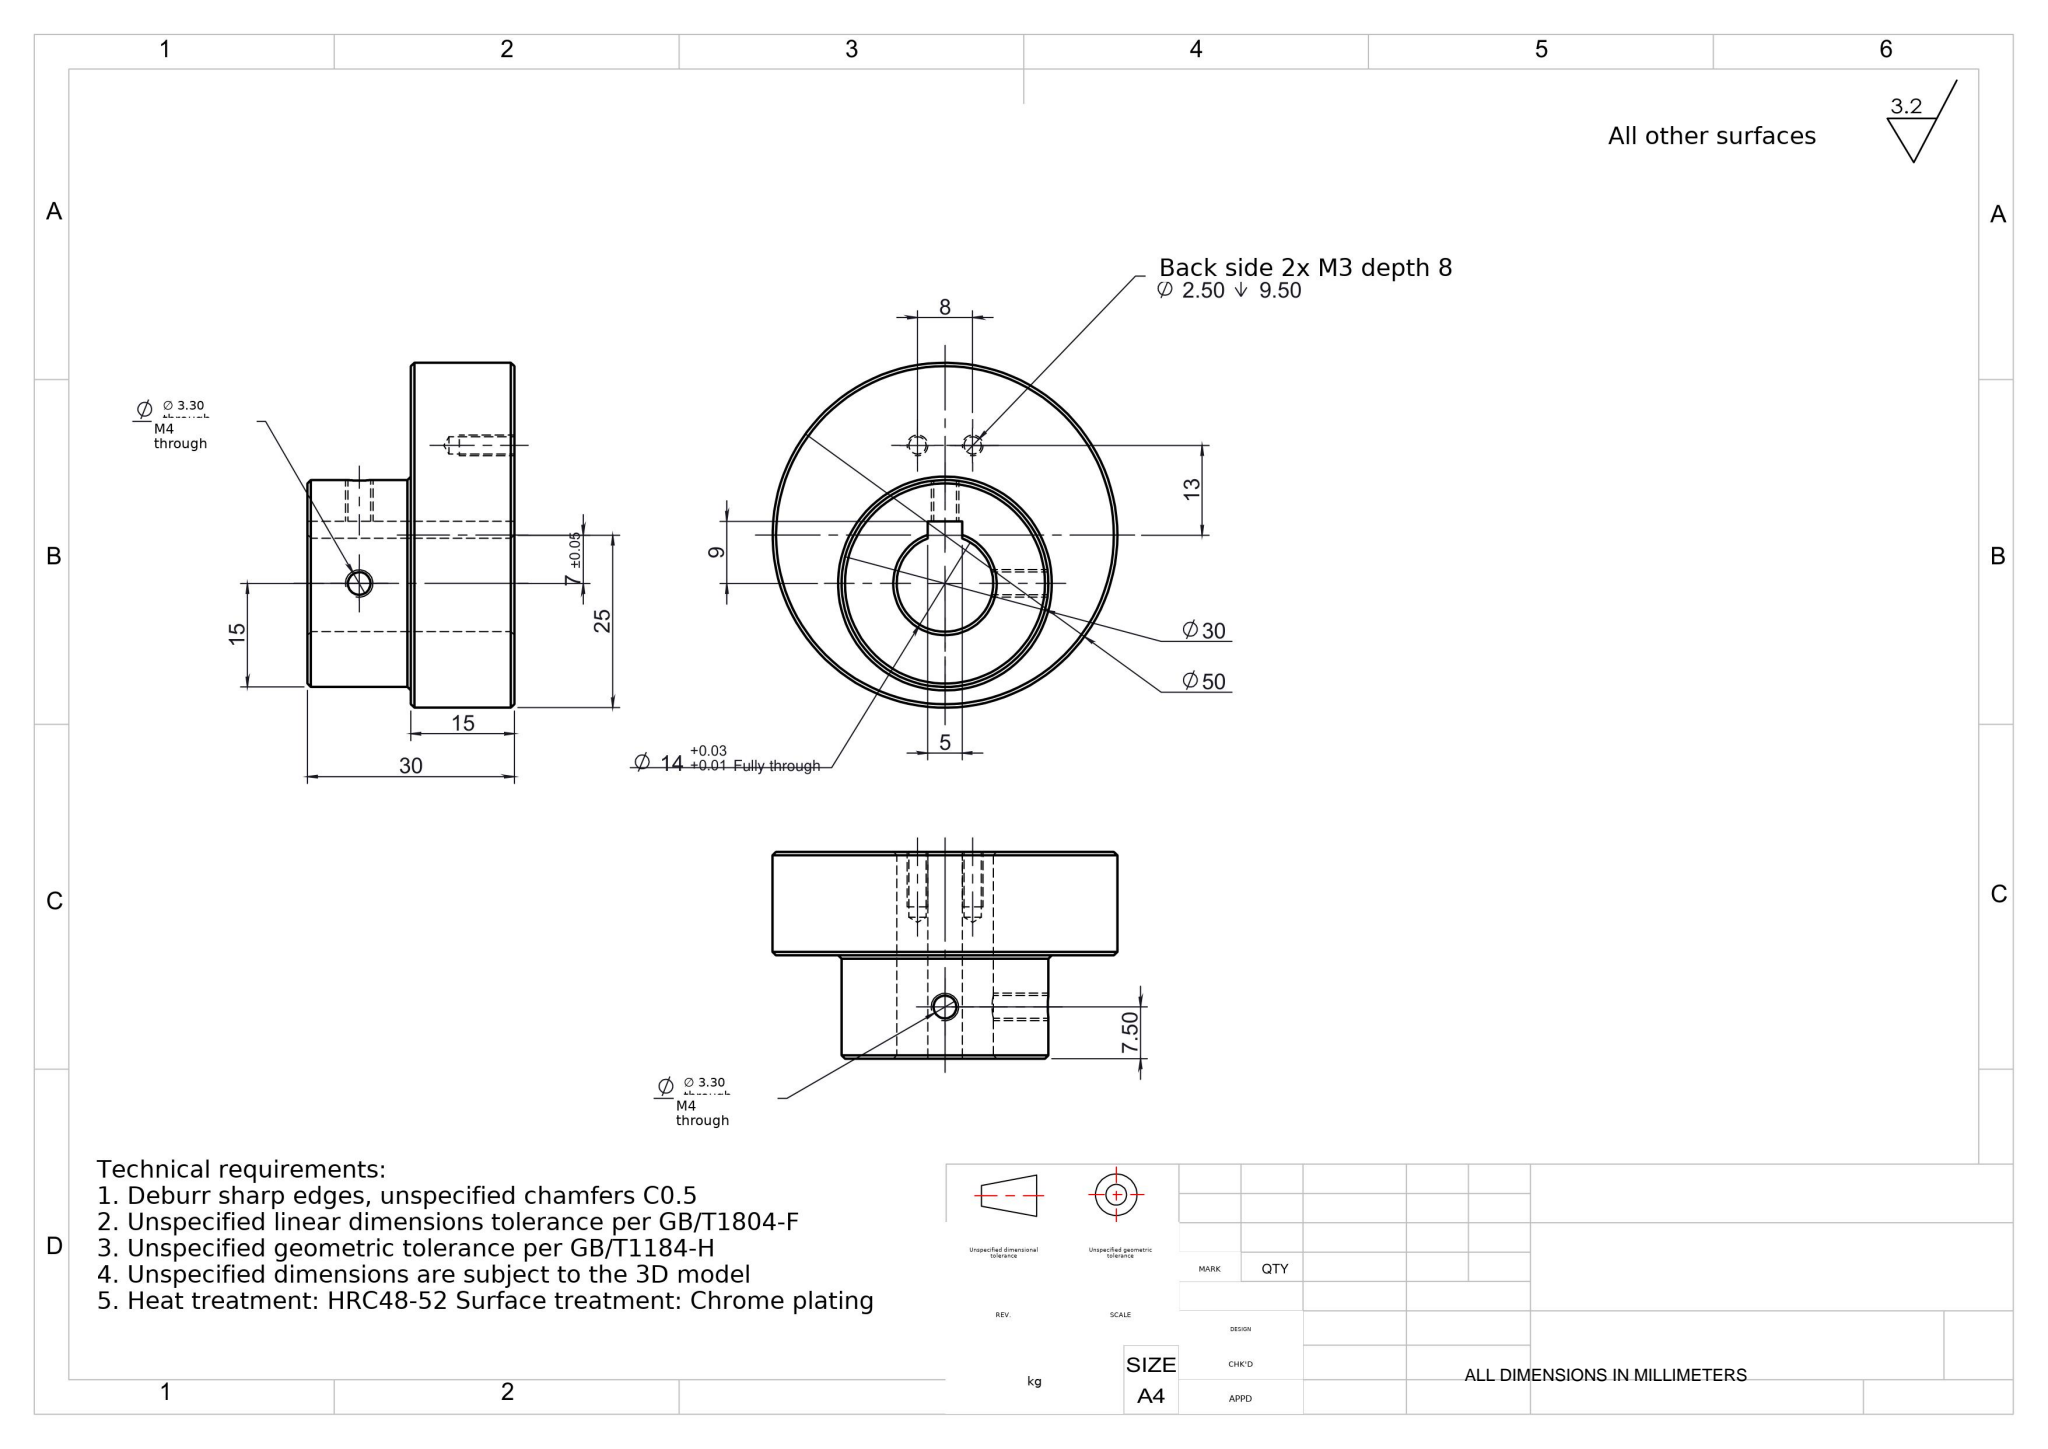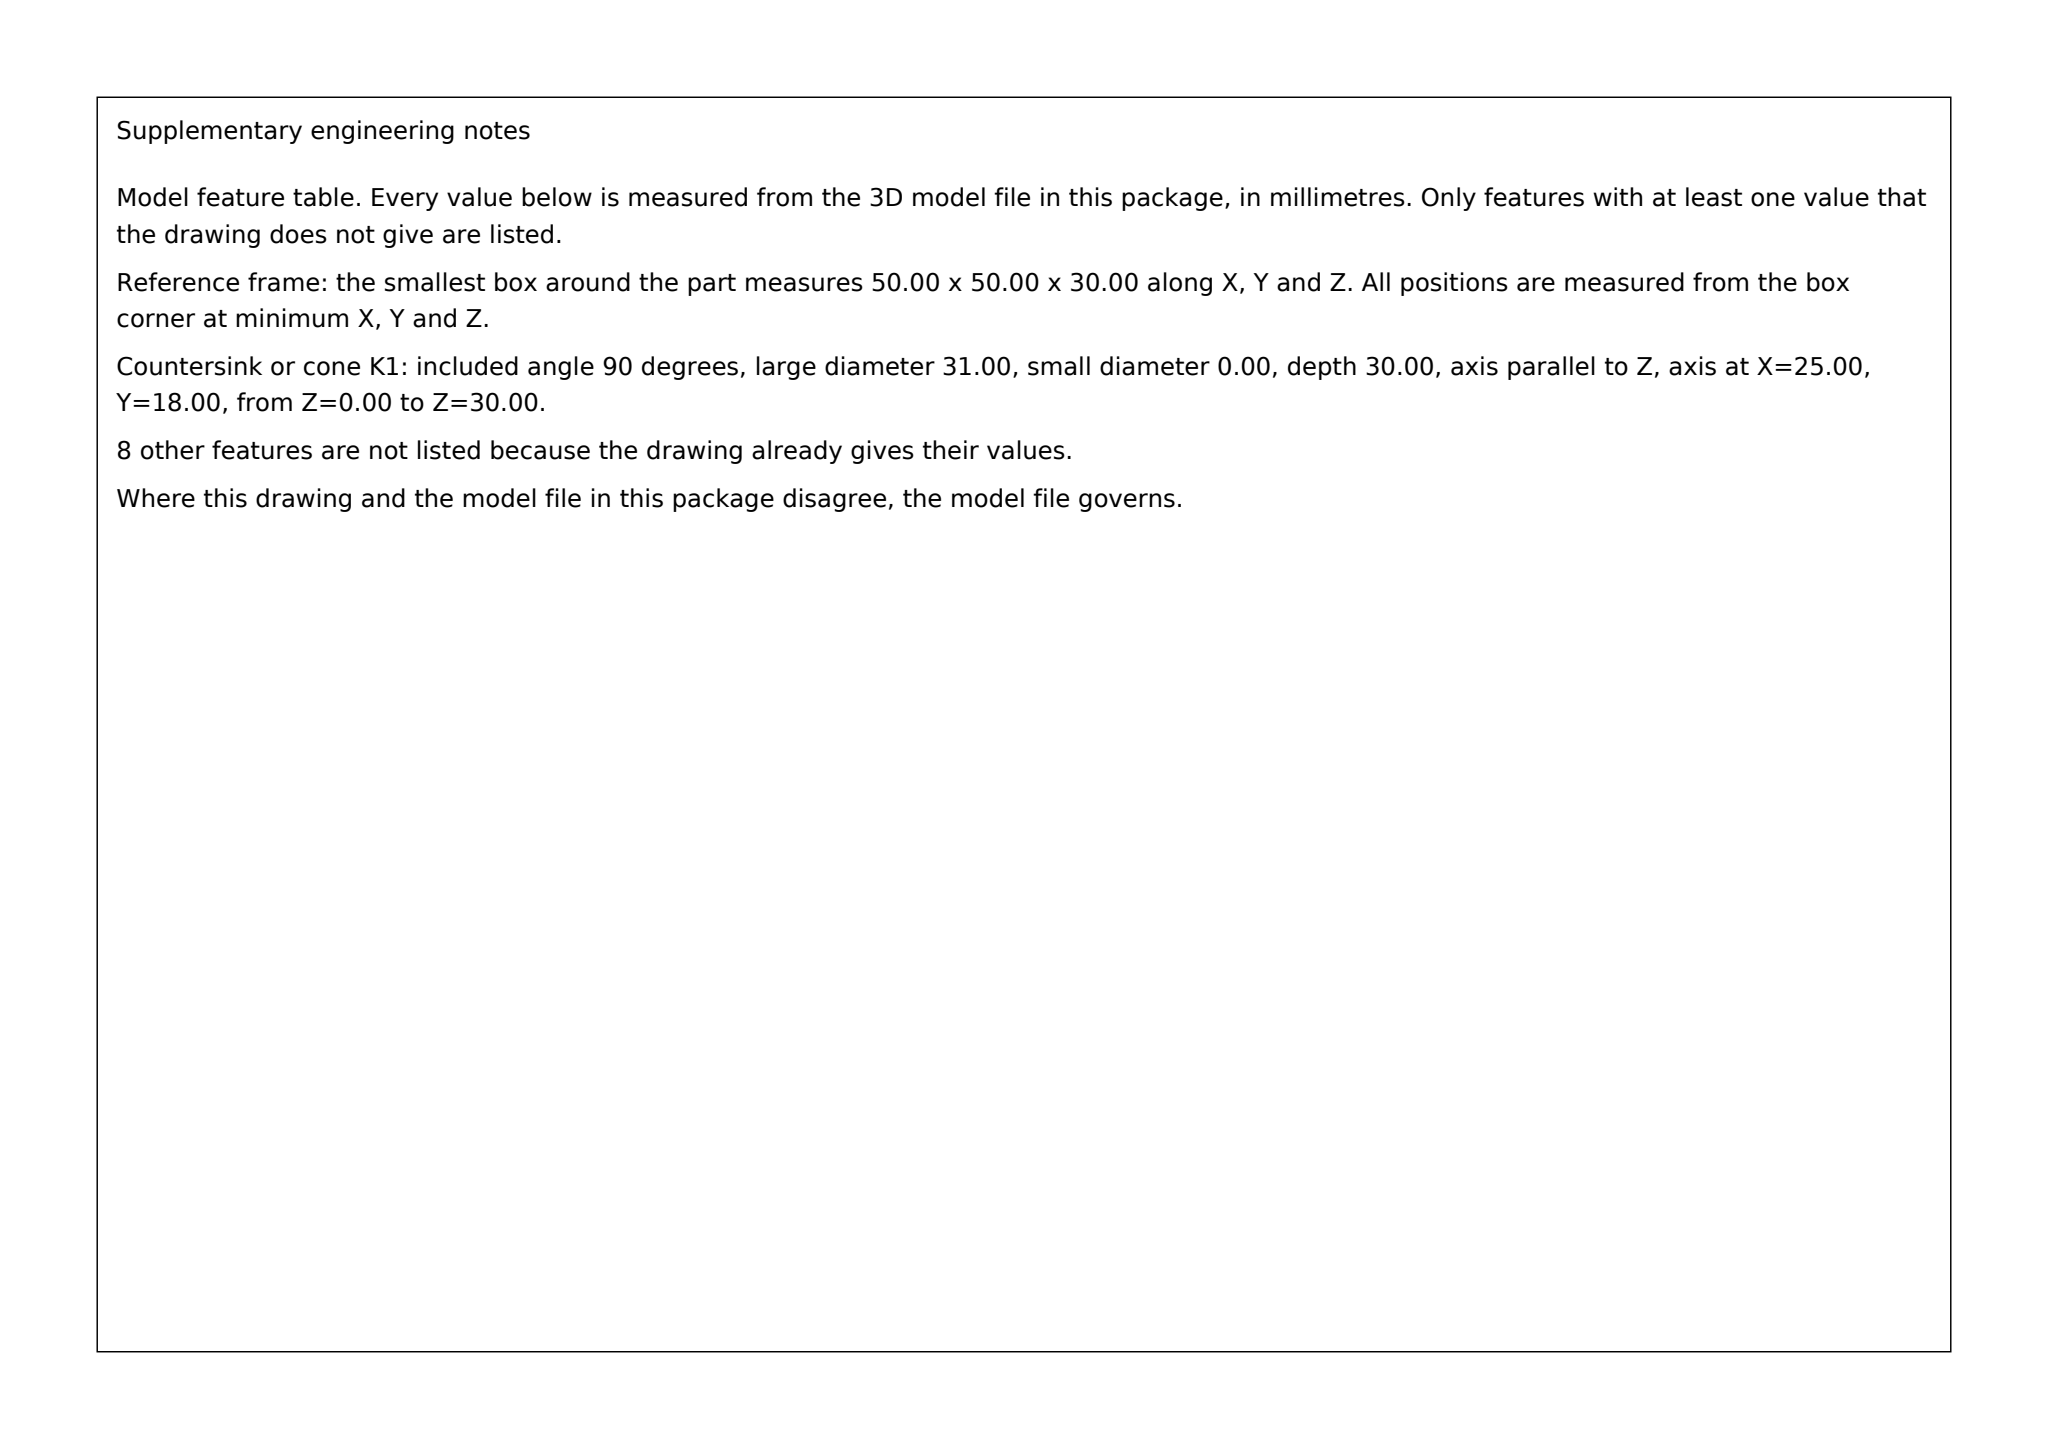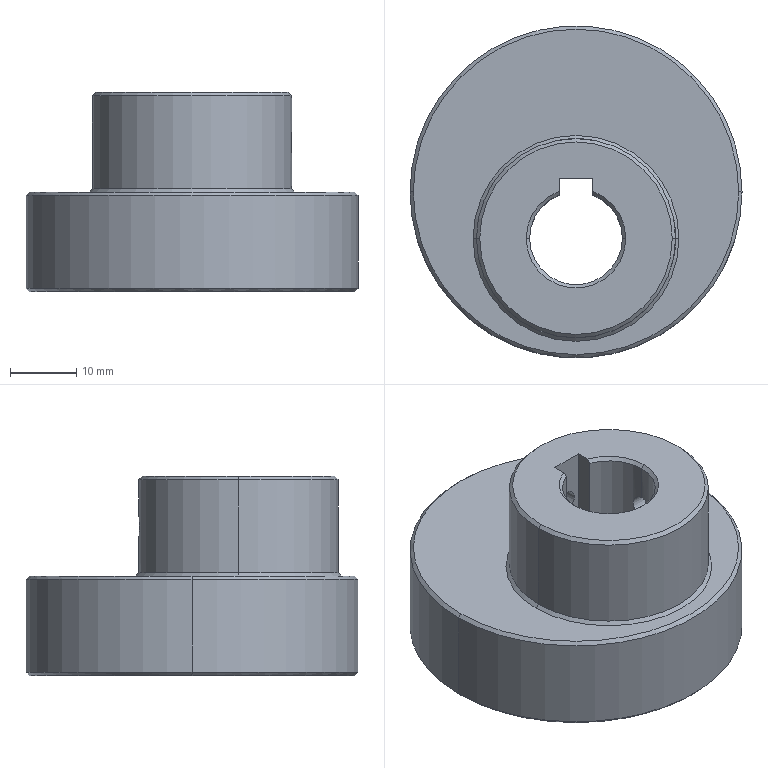Part | SolidWorks | mm | 1 solid | 39 faces | box 50 x 50 x 30 mm | volume 34850 mm3 | cone 18 | cylinder 15 | plane 6 | commonest cylinder face diameters 3.3 x4 2.5 x4 14 x3 30 x2 50 x2
build123d program:
from build123d import *

# Parameters (mm, degrees)
SKETCH1_R                  = 25
BOSS_EXTRUDE1_DEPTH        = 15
F_14_0_14_DIAMETER_HOLE1_D = 14
CHAMFER2_SIZE              = 0.5
M3_TAPPED_HOLE1_D          = 2.5
M3_TAPPED_HOLE1_DEPTH      = 9.5
M3_TAPPED_HOLE1_TIP        = 0.7511
SKETCH15_R                 = 47.133
SKETCH15_R_2               = 15
CUT_EXTRUDE3_DEPTH         = 15
CHAMFER1_SIZE              = 0.5
SKETCH16_W                 = 5
SKETCH16_H                 = 8.591
CUT_EXTRUDE4_DEPTH         = 47.368
M4_TAPPED_HOLE1_D          = 3.3
M4_TAPPED_HOLE1_DEPTH      = 6
M4_TAPPED_HOLE2_REACH      = 51.497
M4_TAPPED_HOLE2_BORE_R     = 1.65


with BuildPart() as part:
    # Sketch1 → Boss-Extrude1 (new, symmetric)
    with BuildSketch(Plane.XY):
        Circle(SKETCH1_R)
    extrude(amount=BOSS_EXTRUDE1_DEPTH, both=True)

    # 14.0 _14_ Diameter Hole1 (through all)
    with Locations(Plane.XY.offset(15)):
        with Locations((0, -7)):
            Hole(F_14_0_14_DIAMETER_HOLE1_D / 2)

    # Chamfer2
    chamfer2_edges = [part.edges().sort_by_distance(p)[0] for p in [
        (7, -7, 15),
        (7, -7, -15),
    ]]
    chamfer(chamfer2_edges, length=CHAMFER2_SIZE)

    # M3 Tapped Hole1
    with Locations(Plane(origin=(0, 0, -15), x_dir=(-1, 0, 0), z_dir=(0, 0, -1))):
        with Locations((4, 13), (-4, 13)):
            Hole(M3_TAPPED_HOLE1_D / 2, depth=M3_TAPPED_HOLE1_DEPTH)
            with Locations((0, 0, -(M3_TAPPED_HOLE1_DEPTH + M3_TAPPED_HOLE1_TIP / 2))):  # 118° drill point
                Cone(0, M3_TAPPED_HOLE1_D / 2, M3_TAPPED_HOLE1_TIP, mode=Mode.SUBTRACT)

    # Sketch15 → Cut-Extrude3 (cut)
    with BuildSketch(Plane.XY.offset(15)):
        with Locations((0, -7)):
            Circle(SKETCH15_R)
        with Locations((0, -7)):
            Circle(SKETCH15_R_2, mode=Mode.SUBTRACT)
    extrude(amount=-CUT_EXTRUDE3_DEPTH, mode=Mode.SUBTRACT)

    # Chamfer1
    chamfer1_edges = [part.edges().sort_by_distance(p)[0] for p in [
        (-25, 0, -15),
        (-15, -7, 0),
        (-25, 0, 0),
        (-15, -7, 15),
    ]]
    chamfer(chamfer1_edges, length=CHAMFER1_SIZE)

    # Sketch16 → Cut-Extrude4 (cut, through all)
    with BuildSketch(Plane.XY.offset(15)):
        with Locations((0, -2.295)):
            Rectangle(SKETCH16_W, SKETCH16_H)
    extrude(amount=-CUT_EXTRUDE4_DEPTH, mode=Mode.SUBTRACT)

    # M4 Tapped Hole1
    with Locations(Plane(origin=(0, 8, 0), x_dir=(1, 0, 0), z_dir=(0, 1, 0))):
        with Locations((0, -7.5)):
            Hole(M4_TAPPED_HOLE1_D / 2, depth=M4_TAPPED_HOLE1_DEPTH)

    # M4 Tapped Hole2 bore → M4 Tapped Hole2 (cut, up to next)
    with BuildSketch(Plane(origin=(15, 0, 0), x_dir=(0, 0, -1), z_dir=(1, 0, 0)), mode=Mode.PRIVATE) as m4_tapped_hole2_sk1:
        with Locations((-7.5, -7)):
            Circle(M4_TAPPED_HOLE2_BORE_R)
    m4_tapped_hole2_tool1 = extrude(m4_tapped_hole2_sk1.sketch, amount=-M4_TAPPED_HOLE2_REACH, mode=Mode.PRIVATE) & part.part
    add(m4_tapped_hole2_tool1.solids().sort_by_distance((15, -7, 7.5))[0], mode=Mode.SUBTRACT)


solid = part.part